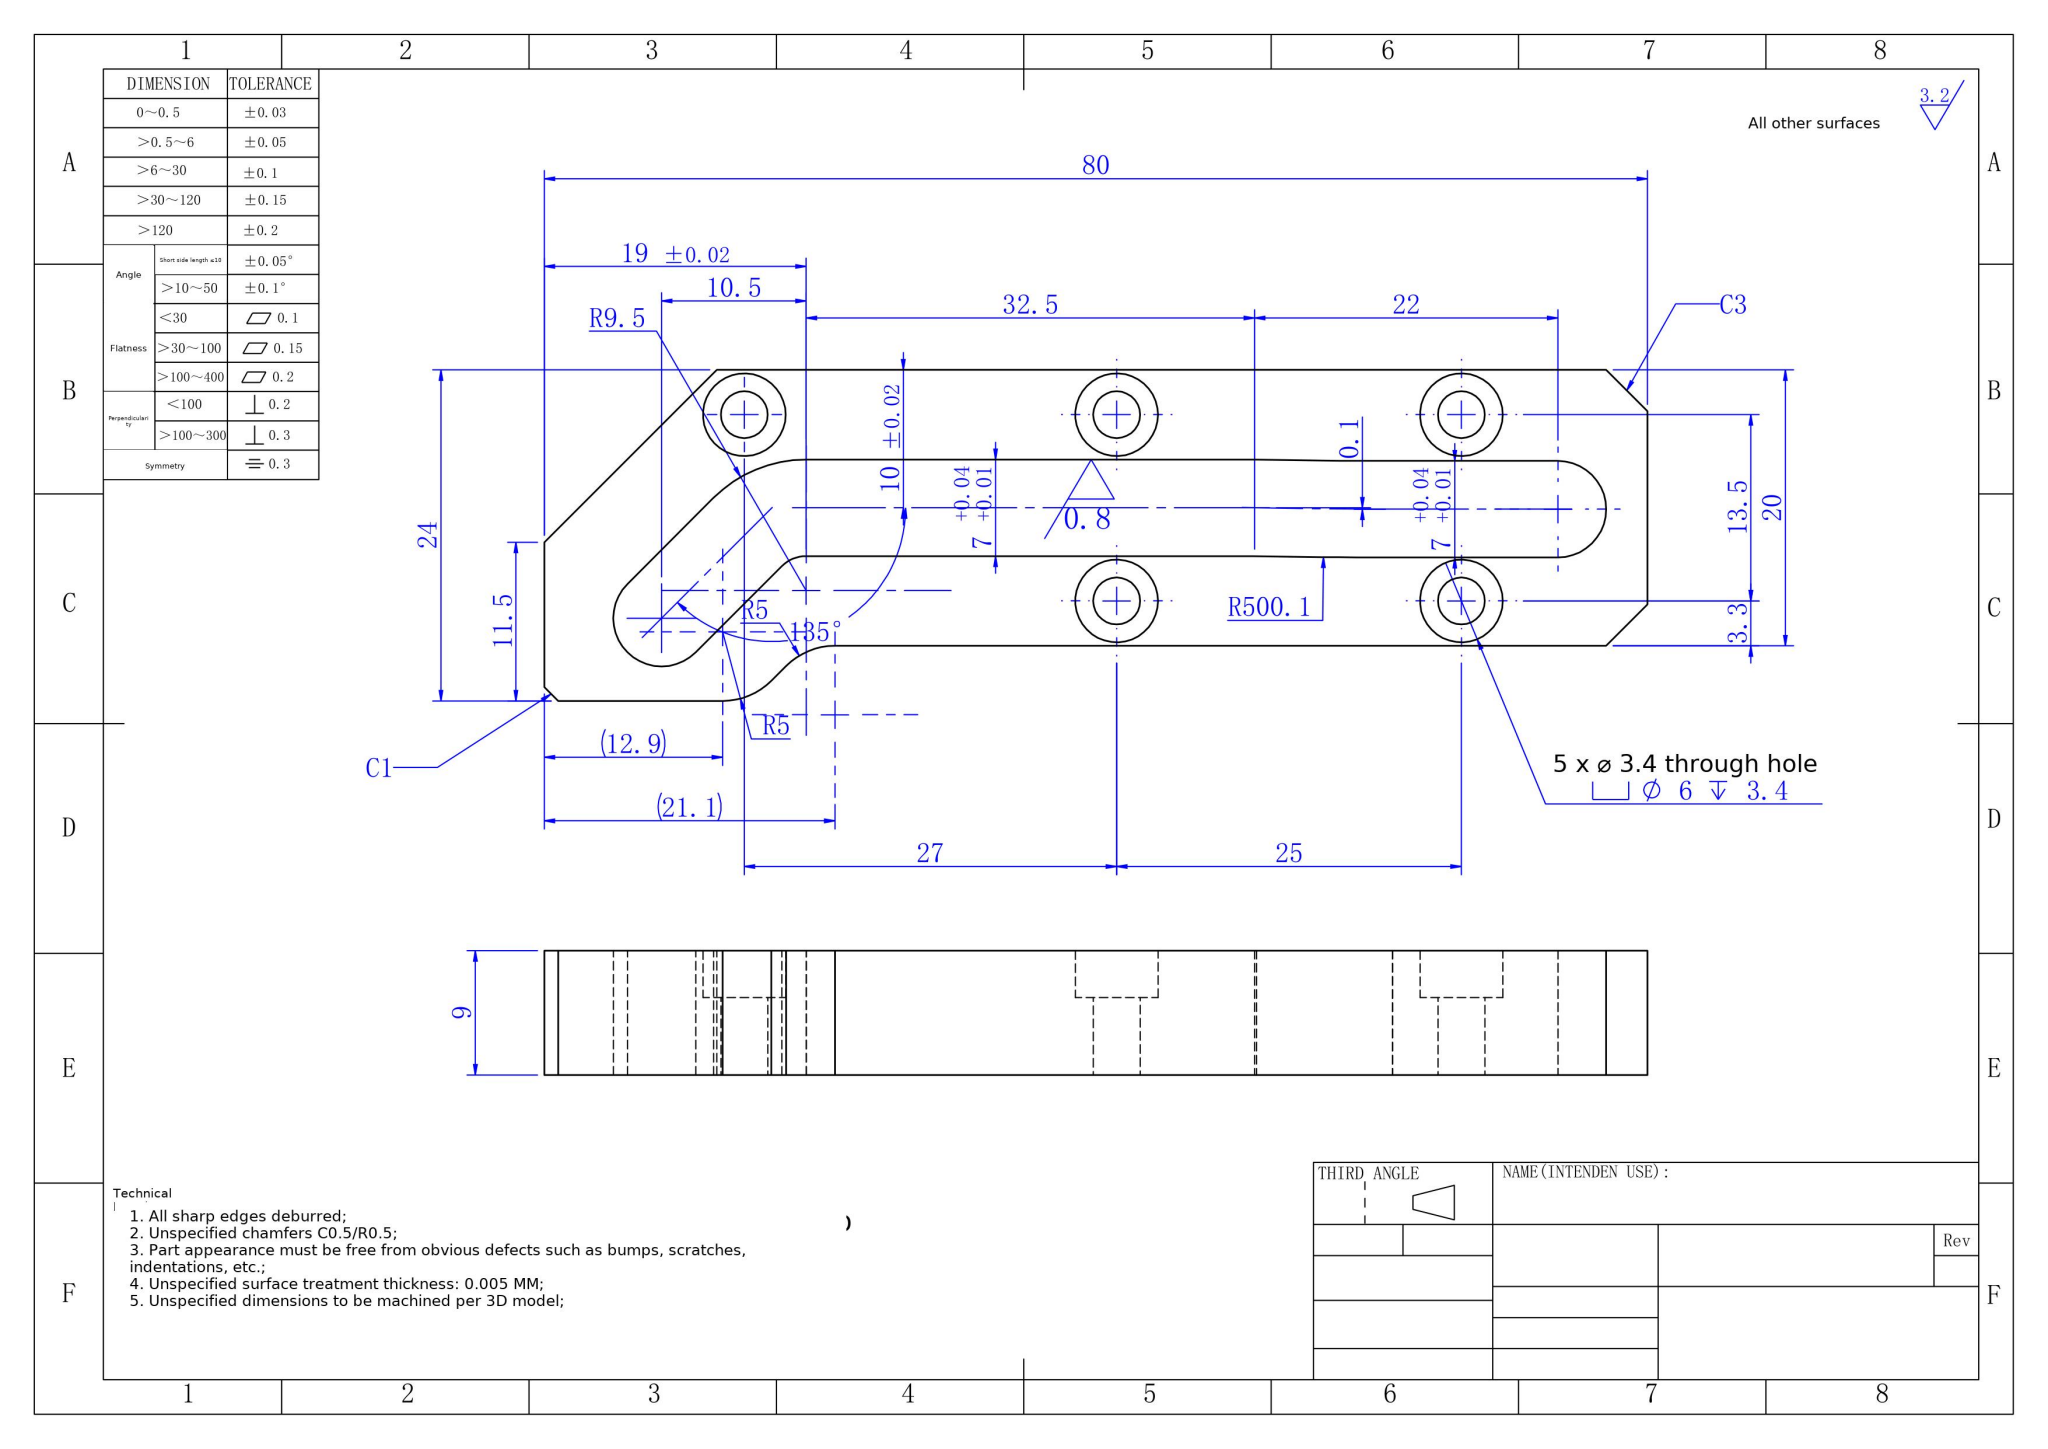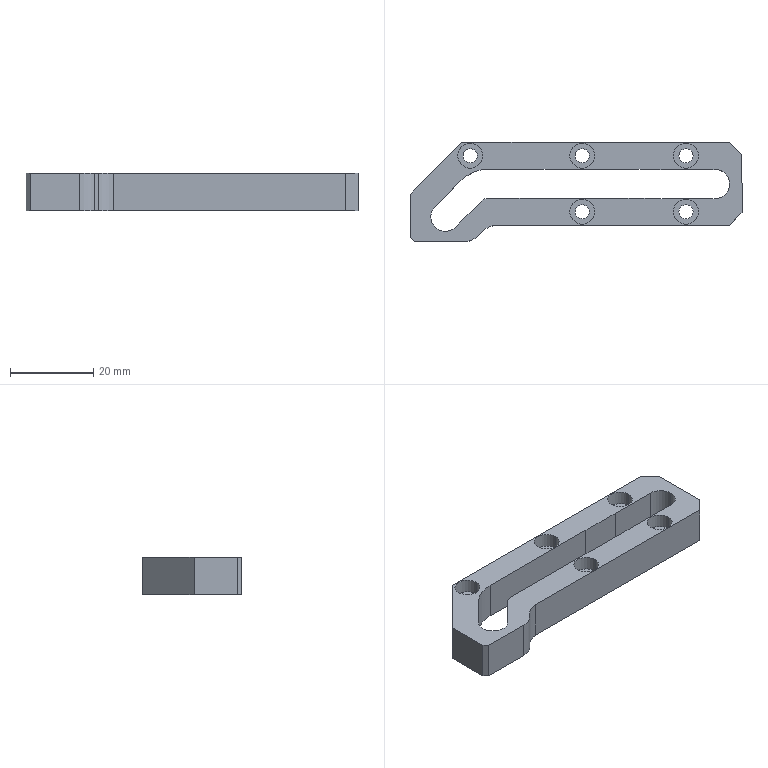Part | SolidWorks | mm | 1 solid | 54 faces | box 80 x 24 x 9 mm | volume 8855 mm3 | cylinder 30 | plane 24 | commonest cylinder face diameters 6 x10 3.4 x10 7 x4 10 x2 19 x1 5 x1 1000.1 x1 986.1 x1